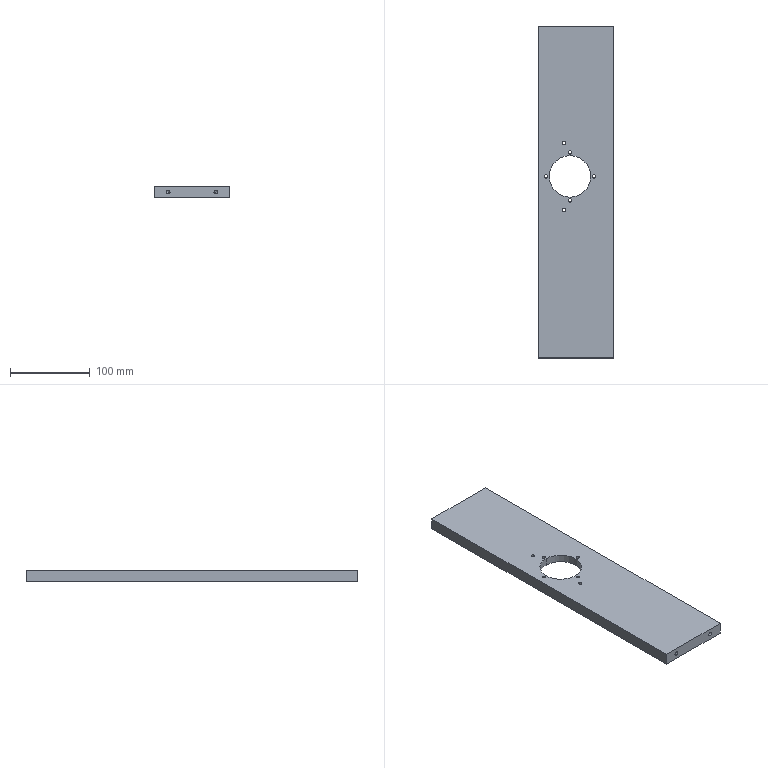Component | SolidWorks | 8TC-A15004-D0-09A-1 | 1 solid | 67 faces | box 95 x 415 x 15 mm | volume 542053 mm3 | cylinder 36 | cone 16 | plane 15 | commonest cylinder face diameters 5 x20 4.2 x12 73 x2 52 x2 | material #45
build123d program:
from build123d import *

# Parameters (mm, degrees)
SKETCH1_W             = 95
SKETCH1_H             = 415
BOSS_EXTRUDE1_DEPTH   = 7.5
SKETCH3_R             = 26
CUT_EXTRUDE2_DEPTH    = 214.395
SKETCH4_R             = 36.5
CUT_EXTRUDE3_DEPTH    = 5
M6_TAPPED_HOLE1_D     = 5
M6_TAPPED_HOLE1_DEPTH = 15
M6_TAPPED_HOLE1_TIP   = 1.502
M6_TAPPED_HOLE2_D     = 5
M6_TAPPED_HOLE2_DEPTH = 15
M6_TAPPED_HOLE2_TIP   = 1.502
M5_TAPPED_HOLE1_D     = 4.2
CIRPATTERN1_COUNT     = 4
M6_TAPPED_HOLE3_D     = 5
M6_TAPPED_HOLE3_DEPTH = 15
M6_TAPPED_HOLE3_TIP   = 1.502
M6_TAPPED_HOLE4_D     = 5
M6_TAPPED_HOLE4_DEPTH = 17
M6_TAPPED_HOLE4_TIP   = 1.502
SKETCH15_W            = 25
SKETCH15_H            = 130
CUT_EXTRUDE4_DEPTH    = 2.5
M5_TAPPED_HOLE2_D     = 4.2
FILLET1_R             = 2.5


with BuildPart() as part:
    # Sketch1 → Boss-Extrude1 (new, symmetric)
    with BuildSketch(Plane(origin=(0, 0, 0), x_dir=(1, 0, 0), z_dir=(0, 1, 0))):
        Rectangle(SKETCH1_W, SKETCH1_H)
    extrude(amount=BOSS_EXTRUDE1_DEPTH, both=True)

    # Sketch3 → Cut-Extrude2 (cut, through all)
    with BuildSketch(Plane.XZ.offset(7.5)):
        with Locations(Location((-7.5, -19.5, 0), (0, 0, 270))):
            Circle(SKETCH3_R)
    extrude(amount=-CUT_EXTRUDE2_DEPTH, mode=Mode.SUBTRACT)

    # Sketch4 → Cut-Extrude3 (cut)
    with BuildSketch(Plane.XZ.offset(7.5)):
        with Locations(Location((-7.5, -19.5, 0), (0, 0, 270))):
            Circle(SKETCH4_R)
    extrude(amount=-CUT_EXTRUDE3_DEPTH, mode=Mode.SUBTRACT)

    # M6 Tapped Hole1
    with Locations(Plane(origin=(0, 0, -207.5), x_dir=(-1, 0, 0), z_dir=(0, 0, -1))):
        with Locations((-30, 0), (30, 0)):
            Hole(M6_TAPPED_HOLE1_D / 2, depth=M6_TAPPED_HOLE1_DEPTH)
            with Locations((0, 0, -(M6_TAPPED_HOLE1_DEPTH + M6_TAPPED_HOLE1_TIP / 2))):  # 118° drill point
                Cone(0, M6_TAPPED_HOLE1_D / 2, M6_TAPPED_HOLE1_TIP, mode=Mode.SUBTRACT)

    # M6 Tapped Hole2
    with Locations(Plane.XY.offset(207.5)):
        with Locations((-30, 0), (30, 0)):
            Hole(M6_TAPPED_HOLE2_D / 2, depth=M6_TAPPED_HOLE2_DEPTH)
            with Locations((0, 0, -(M6_TAPPED_HOLE2_DEPTH + M6_TAPPED_HOLE2_TIP / 2))):  # 118° drill point
                Cone(0, M6_TAPPED_HOLE2_D / 2, M6_TAPPED_HOLE2_TIP, mode=Mode.SUBTRACT)

    # M5 Tapped Hole1 (through all)
    with Locations(Plane(origin=(0, -2.5, 0), x_dir=(-1, 0, 0), z_dir=(0, -1, 0))):
        with Locations((7.5, -10.5)):
            m5_tapped_hole1 = Hole(M5_TAPPED_HOLE1_D / 2)

    # CirPattern1: M5 Tapped Hole1 ×4 about axis
    cirpattern1_axis = Axis((-7.5, 0, -19.5), (0, 1, 0))
    for i in range(1, CIRPATTERN1_COUNT):
        add(m5_tapped_hole1.rotate(cirpattern1_axis, i * 360 / CIRPATTERN1_COUNT), mode=Mode.SUBTRACT)

    # M6 Tapped Hole3
    with Locations(Plane(origin=(47.5, 0, 0), x_dir=(0, 0, -1), z_dir=(1, 0, 0))):
        with Locations((190.5, 0), (140.5, 0)):
            Hole(M6_TAPPED_HOLE3_D / 2, depth=M6_TAPPED_HOLE3_DEPTH)
            with Locations((0, 0, -(M6_TAPPED_HOLE3_DEPTH + M6_TAPPED_HOLE3_TIP / 2))):  # 118° drill point
                Cone(0, M6_TAPPED_HOLE3_D / 2, M6_TAPPED_HOLE3_TIP, mode=Mode.SUBTRACT)

    # M6 Tapped Hole4
    with Locations(Plane(origin=(47.5, 0, 0), x_dir=(0, 0, -1), z_dir=(1, 0, 0))):
        with Locations((175.5, 0), (125.5, 0)):
            Hole(M6_TAPPED_HOLE4_D / 2, depth=M6_TAPPED_HOLE4_DEPTH)
            with Locations((0, 0, -(M6_TAPPED_HOLE4_DEPTH + M6_TAPPED_HOLE4_TIP / 2))):  # 118° drill point
                Cone(0, M6_TAPPED_HOLE4_D / 2, M6_TAPPED_HOLE4_TIP, mode=Mode.SUBTRACT)

    # Sketch15 → Cut-Extrude4 (cut)
    with BuildSketch(Plane.XZ.offset(7.5)):
        with Locations((-15, -19.5)):
            Rectangle(SKETCH15_W, SKETCH15_H)
    extrude(amount=-CUT_EXTRUDE4_DEPTH, mode=Mode.SUBTRACT)

    # M5 Tapped Hole2 (through all)
    with Locations(Plane(origin=(0, -5, 0), x_dir=(-1, 0, 0), z_dir=(0, -1, 0))):
        with Locations((15, -22.5), (15, 61.5)):
            Hole(M5_TAPPED_HOLE2_D / 2)

    # Fillet1
    fillet1_edges = [part.edges().sort_by_distance(p)[0] for p in [
        (-2.5, -6.25, 45.5),
        (-27.5, -6.25, -84.5),
        (-2.5, -6.25, -84.5),
        (-27.5, -6.25, 45.5),
    ]]
    fillet(fillet1_edges, radius=FILLET1_R)


solid = part.part

# Placed as in the assembly
solid = solid.moved(Location((0, 215, -117.5), (90, 0, 0)))